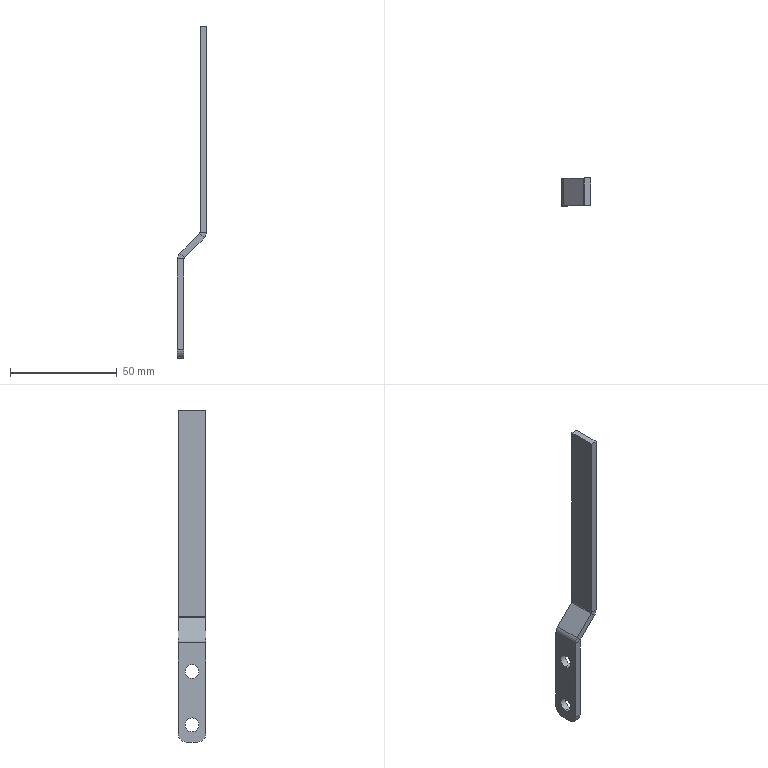Component | SolidWorks | GlassDoorAssembly-1_828LockAssembly-1_UpperPullRod-1 | 1 solid | 28 faces | box 13.61 x 13 x 155.61 mm | volume 6013 mm3 | plane 18 | cylinder 10 | commonest cylinder face diameters 6.5 x4 7.473 x2 1.473 x2 8 x2
STEP:
#1=COLOUR_RGB('',0.7922,0.8196,0.9333);
#2=FILL_AREA_STYLE_COLOUR('',#1);
#3=FILL_AREA_STYLE('',(#2));
#4=SURFACE_STYLE_FILL_AREA(#3);
#5=SURFACE_SIDE_STYLE('',(#4));
#6=SURFACE_STYLE_USAGE(.BOTH.,#5);
#7=PRESENTATION_STYLE_ASSIGNMENT((#6));
#8=CARTESIAN_POINT('',(-16.306,-19.747,-36.852));
#9=VERTEX_POINT('',#8);
#10=CARTESIAN_POINT('',(-16.306,-19.747,-36.596));
#11=VERTEX_POINT('',#10);
#12=CARTESIAN_POINT('',(-16.306,-19.747,-36.724));
#13=DIRECTION('',(1.,0.,0.));
#14=DIRECTION('',(0.,0.,1.));
#15=AXIS2_PLACEMENT_3D('',#12,#13,#14);
#16=CIRCLE('',#15,0.128);
#17=EDGE_CURVE('',#9,#11,#16,.T.);
#18=ORIENTED_EDGE('',*,*,#17,.F.);
#19=CARTESIAN_POINT('',(-16.188,-19.747,-36.852));
#20=VERTEX_POINT('',#19);
#21=CARTESIAN_POINT('',(-16.306,-19.747,-36.852));
#22=DIRECTION('',(1.,0.,0.));
#23=VECTOR('',#22,39.37);
#24=LINE('',#21,#23);
#25=EDGE_CURVE('',#9,#20,#24,.T.);
#26=ORIENTED_EDGE('',*,*,#25,.T.);
#27=CARTESIAN_POINT('',(-16.188,-19.747,-36.596));
#28=VERTEX_POINT('',#27);
#29=CARTESIAN_POINT('',(-16.188,-19.747,-36.724));
#30=DIRECTION('',(1.,0.,0.));
#31=DIRECTION('',(0.,0.,1.));
#32=AXIS2_PLACEMENT_3D('',#29,#30,#31);
#33=CIRCLE('',#32,0.128);
#34=EDGE_CURVE('',#20,#28,#33,.T.);
#35=ORIENTED_EDGE('',*,*,#34,.T.);
#36=CARTESIAN_POINT('',(-16.306,-19.747,-36.596));
#37=DIRECTION('',(1.,0.,0.));
#38=VECTOR('',#37,39.37);
#39=LINE('',#36,#38);
#40=EDGE_CURVE('',#11,#28,#39,.T.);
#41=ORIENTED_EDGE('',*,*,#40,.F.);
#42=EDGE_LOOP('',(#18,#26,#35,#41));
#43=FACE_OUTER_BOUND('',#42,.T.);
#44=CARTESIAN_POINT('',(-16.306,-19.747,-36.724));
#45=DIRECTION('',(1.,0.,0.));
#46=DIRECTION('',(0.,0.,1.));
#47=AXIS2_PLACEMENT_3D('',#44,#45,#46);
#48=CYLINDRICAL_SURFACE('',#47,0.128);
#49=ADVANCED_FACE('',(#43),#48,.F.);
#50=CARTESIAN_POINT('',(-16.306,-19.747,-37.836));
#51=VERTEX_POINT('',#50);
#52=CARTESIAN_POINT('',(-16.306,-19.747,-37.58));
#53=VERTEX_POINT('',#52);
#54=CARTESIAN_POINT('',(-16.306,-19.747,-37.708));
#55=DIRECTION('',(1.,0.,0.));
#56=DIRECTION('',(0.,0.,1.));
#57=AXIS2_PLACEMENT_3D('',#54,#55,#56);
#58=CIRCLE('',#57,0.128);
#59=EDGE_CURVE('',#51,#53,#58,.T.);
#60=ORIENTED_EDGE('',*,*,#59,.F.);
#61=CARTESIAN_POINT('',(-16.188,-19.747,-37.836));
#62=VERTEX_POINT('',#61);
#63=CARTESIAN_POINT('',(-16.306,-19.747,-37.836));
#64=DIRECTION('',(1.,0.,0.));
#65=VECTOR('',#64,39.37);
#66=LINE('',#63,#65);
#67=EDGE_CURVE('',#51,#62,#66,.T.);
#68=ORIENTED_EDGE('',*,*,#67,.T.);
#69=CARTESIAN_POINT('',(-16.188,-19.747,-37.58));
#70=VERTEX_POINT('',#69);
#71=CARTESIAN_POINT('',(-16.188,-19.747,-37.708));
#72=DIRECTION('',(1.,0.,0.));
#73=DIRECTION('',(0.,0.,1.));
#74=AXIS2_PLACEMENT_3D('',#71,#72,#73);
#75=CIRCLE('',#74,0.128);
#76=EDGE_CURVE('',#62,#70,#75,.T.);
#77=ORIENTED_EDGE('',*,*,#76,.T.);
#78=CARTESIAN_POINT('',(-16.306,-19.747,-37.58));
#79=DIRECTION('',(1.,0.,0.));
#80=VECTOR('',#79,39.37);
#81=LINE('',#78,#80);
#82=EDGE_CURVE('',#53,#70,#81,.T.);
#83=ORIENTED_EDGE('',*,*,#82,.F.);
#84=EDGE_LOOP('',(#60,#68,#77,#83));
#85=FACE_OUTER_BOUND('',#84,.T.);
#86=CARTESIAN_POINT('',(-16.306,-19.747,-37.708));
#87=DIRECTION('',(1.,0.,0.));
#88=DIRECTION('',(0.,0.,1.));
#89=AXIS2_PLACEMENT_3D('',#86,#87,#88);
#90=CYLINDRICAL_SURFACE('',#89,0.128);
#91=ADVANCED_FACE('',(#85),#90,.F.);
#92=CARTESIAN_POINT('',(-16.18,-19.491,-36.174));
#93=VERTEX_POINT('',#92);
#94=CARTESIAN_POINT('',(-16.263,-19.491,-36.09));
#95=VERTEX_POINT('',#94);
#96=CARTESIAN_POINT('',(-16.18,-19.491,-36.174));
#97=DIRECTION('',(-0.7071,-0.,0.7071));
#98=VECTOR('',#97,39.37);
#99=LINE('',#96,#98);
#100=EDGE_CURVE('',#93,#95,#99,.T.);
#101=ORIENTED_EDGE('',*,*,#100,.T.);
#102=CARTESIAN_POINT('',(-15.897,-19.491,-35.724));
#103=VERTEX_POINT('',#102);
#104=CARTESIAN_POINT('',(-15.889,-19.491,-35.716));
#105=DIRECTION('',(0.7071,0.,0.7071));
#106=VECTOR('',#105,39.37);
#107=LINE('',#104,#106);
#108=EDGE_CURVE('',#95,#103,#107,.T.);
#109=ORIENTED_EDGE('',*,*,#108,.T.);
#110=CARTESIAN_POINT('',(-15.814,-19.491,-35.808));
#111=VERTEX_POINT('',#110);
#112=CARTESIAN_POINT('',(-15.897,-19.491,-35.724));
#113=DIRECTION('',(0.7071,0.,-0.7071));
#114=VECTOR('',#113,39.37);
#115=LINE('',#112,#114);
#116=EDGE_CURVE('',#103,#111,#115,.T.);
#117=ORIENTED_EDGE('',*,*,#116,.T.);
#118=CARTESIAN_POINT('',(-15.805,-19.491,-35.799));
#119=DIRECTION('',(0.7071,0.,0.7071));
#120=VECTOR('',#119,39.37);
#121=LINE('',#118,#120);
#122=EDGE_CURVE('',#93,#111,#121,.T.);
#123=ORIENTED_EDGE('',*,*,#122,.F.);
#124=EDGE_LOOP('',(#101,#109,#117,#123));
#125=FACE_OUTER_BOUND('',#124,.T.);
#126=CARTESIAN_POINT('',(-15.805,-19.491,-35.799));
#127=DIRECTION('',(0.,-1.,-0.));
#128=DIRECTION('',(-1.,-0.,-0.));
#129=AXIS2_PLACEMENT_3D('',#126,#127,#128);
#130=PLANE('',#129);
#131=ADVANCED_FACE('',(#125),#130,.F.);
#132=CARTESIAN_POINT('',(-16.18,-20.003,-36.174));
#133=VERTEX_POINT('',#132);
#134=CARTESIAN_POINT('',(-16.263,-20.003,-36.09));
#135=VERTEX_POINT('',#134);
#136=CARTESIAN_POINT('',(-16.18,-20.003,-36.174));
#137=DIRECTION('',(-0.7071,-0.,0.7071));
#138=VECTOR('',#137,39.37);
#139=LINE('',#136,#138);
#140=EDGE_CURVE('',#133,#135,#139,.T.);
#141=ORIENTED_EDGE('',*,*,#140,.F.);
#142=CARTESIAN_POINT('',(-15.814,-20.003,-35.808));
#143=VERTEX_POINT('',#142);
#144=CARTESIAN_POINT('',(-16.188,-20.003,-36.182));
#145=DIRECTION('',(-0.7071,-0.,-0.7071));
#146=VECTOR('',#145,39.37);
#147=LINE('',#144,#146);
#148=EDGE_CURVE('',#143,#133,#147,.T.);
#149=ORIENTED_EDGE('',*,*,#148,.F.);
#150=CARTESIAN_POINT('',(-15.897,-20.003,-35.724));
#151=VERTEX_POINT('',#150);
#152=CARTESIAN_POINT('',(-15.897,-20.003,-35.724));
#153=DIRECTION('',(0.7071,0.,-0.7071));
#154=VECTOR('',#153,39.37);
#155=LINE('',#152,#154);
#156=EDGE_CURVE('',#151,#143,#155,.T.);
#157=ORIENTED_EDGE('',*,*,#156,.F.);
#158=CARTESIAN_POINT('',(-16.272,-20.003,-36.099));
#159=DIRECTION('',(-0.7071,-0.,-0.7071));
#160=VECTOR('',#159,39.37);
#161=LINE('',#158,#160);
#162=EDGE_CURVE('',#151,#135,#161,.T.);
#163=ORIENTED_EDGE('',*,*,#162,.T.);
#164=EDGE_LOOP('',(#141,#149,#157,#163));
#165=FACE_OUTER_BOUND('',#164,.T.);
#166=CARTESIAN_POINT('',(-16.188,-20.003,-36.182));
#167=DIRECTION('',(-0.,1.,0.));
#168=DIRECTION('',(1.,0.,0.));
#169=AXIS2_PLACEMENT_3D('',#166,#167,#168);
#170=PLANE('',#169);
#171=ADVANCED_FACE('',(#165),#170,.F.);
#172=CARTESIAN_POINT('',(-16.18,-19.491,-36.174));
#173=DIRECTION('',(0.,-1.,-0.));
#174=VECTOR('',#173,39.37);
#175=LINE('',#172,#174);
#176=EDGE_CURVE('',#93,#133,#175,.T.);
#177=ORIENTED_EDGE('',*,*,#176,.F.);
#178=ORIENTED_EDGE('',*,*,#122,.T.);
#179=CARTESIAN_POINT('',(-15.814,-19.491,-35.808));
#180=DIRECTION('',(-0.,1.,0.));
#181=VECTOR('',#180,39.37);
#182=LINE('',#179,#181);
#183=EDGE_CURVE('',#143,#111,#182,.T.);
#184=ORIENTED_EDGE('',*,*,#183,.F.);
#185=ORIENTED_EDGE('',*,*,#148,.T.);
#186=EDGE_LOOP('',(#177,#178,#184,#185));
#187=FACE_OUTER_BOUND('',#186,.T.);
#188=CARTESIAN_POINT('',(-16.188,-19.491,-36.182));
#189=DIRECTION('',(-0.7071,-0.,0.7071));
#190=DIRECTION('',(-0.7071,-0.,-0.7071));
#191=AXIS2_PLACEMENT_3D('',#188,#189,#190);
#192=PLANE('',#191);
#193=ADVANCED_FACE('',(#187),#192,.F.);
#194=ORIENTED_EDGE('',*,*,#108,.F.);
#195=CARTESIAN_POINT('',(-16.263,-19.491,-36.09));
#196=DIRECTION('',(0.,-1.,-0.));
#197=VECTOR('',#196,39.37);
#198=LINE('',#195,#197);
#199=EDGE_CURVE('',#95,#135,#198,.T.);
#200=ORIENTED_EDGE('',*,*,#199,.T.);
#201=ORIENTED_EDGE('',*,*,#162,.F.);
#202=CARTESIAN_POINT('',(-15.897,-19.491,-35.724));
#203=DIRECTION('',(0.,-1.,-0.));
#204=VECTOR('',#203,39.37);
#205=LINE('',#202,#204);
#206=EDGE_CURVE('',#103,#151,#205,.T.);
#207=ORIENTED_EDGE('',*,*,#206,.F.);
#208=EDGE_LOOP('',(#194,#200,#201,#207));
#209=FACE_OUTER_BOUND('',#208,.T.);
#210=CARTESIAN_POINT('',(-16.272,-19.491,-36.099));
#211=DIRECTION('',(-0.7071,-0.,0.7071));
#212=DIRECTION('',(-0.7071,-0.,-0.7071));
#213=AXIS2_PLACEMENT_3D('',#210,#211,#212);
#214=PLANE('',#213);
#215=ADVANCED_FACE('',(#209),#214,.T.);
#216=CARTESIAN_POINT('',(-15.889,-20.003,-35.704));
#217=VERTEX_POINT('',#216);
#218=CARTESIAN_POINT('',(-15.889,-20.003,-31.897));
#219=VERTEX_POINT('',#218);
#220=CARTESIAN_POINT('',(-15.889,-20.003,-31.897));
#221=DIRECTION('',(-0.,-0.,1.));
#222=VECTOR('',#221,39.37);
#223=LINE('',#220,#222);
#224=EDGE_CURVE('',#217,#219,#223,.T.);
#225=ORIENTED_EDGE('',*,*,#224,.F.);
#226=CARTESIAN_POINT('',(-15.771,-20.003,-35.704));
#227=VERTEX_POINT('',#226);
#228=CARTESIAN_POINT('',(-15.889,-20.003,-35.704));
#229=DIRECTION('',(1.,0.,0.));
#230=VECTOR('',#229,39.37);
#231=LINE('',#228,#230);
#232=EDGE_CURVE('',#217,#227,#231,.T.);
#233=ORIENTED_EDGE('',*,*,#232,.T.);
#234=CARTESIAN_POINT('',(-15.771,-20.003,-31.897));
#235=VERTEX_POINT('',#234);
#236=CARTESIAN_POINT('',(-15.771,-20.003,-31.897));
#237=DIRECTION('',(-0.,-0.,1.));
#238=VECTOR('',#237,39.37);
#239=LINE('',#236,#238);
#240=EDGE_CURVE('',#227,#235,#239,.T.);
#241=ORIENTED_EDGE('',*,*,#240,.T.);
#242=CARTESIAN_POINT('',(-15.771,-20.003,-31.897));
#243=DIRECTION('',(-1.,-0.,-0.));
#244=VECTOR('',#243,39.37);
#245=LINE('',#242,#244);
#246=EDGE_CURVE('',#235,#219,#245,.T.);
#247=ORIENTED_EDGE('',*,*,#246,.T.);
#248=EDGE_LOOP('',(#225,#233,#241,#247));
#249=FACE_OUTER_BOUND('',#248,.T.);
#250=CARTESIAN_POINT('',(-15.771,-20.003,-31.897));
#251=DIRECTION('',(0.,-1.,-0.));
#252=DIRECTION('',(-1.,-0.,-0.));
#253=AXIS2_PLACEMENT_3D('',#250,#251,#252);
#254=PLANE('',#253);
#255=ADVANCED_FACE('',(#249),#254,.T.);
#256=CARTESIAN_POINT('',(-15.771,-19.491,-35.704));
#257=VERTEX_POINT('',#256);
#258=CARTESIAN_POINT('',(-15.771,-20.003,-35.704));
#259=DIRECTION('',(-0.,1.,0.));
#260=VECTOR('',#259,39.37);
#261=LINE('',#258,#260);
#262=EDGE_CURVE('',#227,#257,#261,.T.);
#263=ORIENTED_EDGE('',*,*,#262,.T.);
#264=CARTESIAN_POINT('',(-15.771,-19.491,-31.897));
#265=VERTEX_POINT('',#264);
#266=CARTESIAN_POINT('',(-15.771,-19.491,-31.897));
#267=DIRECTION('',(0.,0.,-1.));
#268=VECTOR('',#267,39.37);
#269=LINE('',#266,#268);
#270=EDGE_CURVE('',#265,#257,#269,.T.);
#271=ORIENTED_EDGE('',*,*,#270,.F.);
#272=CARTESIAN_POINT('',(-15.771,-20.003,-31.897));
#273=DIRECTION('',(-0.,1.,0.));
#274=VECTOR('',#273,39.37);
#275=LINE('',#272,#274);
#276=EDGE_CURVE('',#235,#265,#275,.T.);
#277=ORIENTED_EDGE('',*,*,#276,.F.);
#278=ORIENTED_EDGE('',*,*,#240,.F.);
#279=EDGE_LOOP('',(#263,#271,#277,#278));
#280=FACE_OUTER_BOUND('',#279,.T.);
#281=CARTESIAN_POINT('',(-15.771,-19.491,-35.716));
#282=DIRECTION('',(-1.,-0.,-0.));
#283=DIRECTION('',(0.,0.,-1.));
#284=AXIS2_PLACEMENT_3D('',#281,#282,#283);
#285=PLANE('',#284);
#286=ADVANCED_FACE('',(#280),#285,.F.);
#287=CARTESIAN_POINT('',(-15.889,-19.491,-31.897));
#288=VERTEX_POINT('',#287);
#289=CARTESIAN_POINT('',(-15.889,-19.491,-35.704));
#290=VERTEX_POINT('',#289);
#291=CARTESIAN_POINT('',(-15.889,-19.491,-31.897));
#292=DIRECTION('',(0.,0.,-1.));
#293=VECTOR('',#292,39.37);
#294=LINE('',#291,#293);
#295=EDGE_CURVE('',#288,#290,#294,.T.);
#296=ORIENTED_EDGE('',*,*,#295,.T.);
#297=CARTESIAN_POINT('',(-15.889,-20.003,-35.704));
#298=DIRECTION('',(-0.,1.,0.));
#299=VECTOR('',#298,39.37);
#300=LINE('',#297,#299);
#301=EDGE_CURVE('',#217,#290,#300,.T.);
#302=ORIENTED_EDGE('',*,*,#301,.F.);
#303=ORIENTED_EDGE('',*,*,#224,.T.);
#304=CARTESIAN_POINT('',(-15.889,-20.003,-31.897));
#305=DIRECTION('',(-0.,1.,0.));
#306=VECTOR('',#305,39.37);
#307=LINE('',#304,#306);
#308=EDGE_CURVE('',#219,#288,#307,.T.);
#309=ORIENTED_EDGE('',*,*,#308,.T.);
#310=EDGE_LOOP('',(#296,#302,#303,#309));
#311=FACE_OUTER_BOUND('',#310,.T.);
#312=CARTESIAN_POINT('',(-15.889,-19.491,-35.716));
#313=DIRECTION('',(-1.,-0.,-0.));
#314=DIRECTION('',(0.,0.,-1.));
#315=AXIS2_PLACEMENT_3D('',#312,#313,#314);
#316=PLANE('',#315);
#317=ADVANCED_FACE('',(#311),#316,.T.);
#318=CARTESIAN_POINT('',(-15.889,-19.491,-35.704));
#319=DIRECTION('',(1.,0.,0.));
#320=VECTOR('',#319,39.37);
#321=LINE('',#318,#320);
#322=EDGE_CURVE('',#290,#257,#321,.T.);
#323=ORIENTED_EDGE('',*,*,#322,.F.);
#324=ORIENTED_EDGE('',*,*,#295,.F.);
#325=CARTESIAN_POINT('',(-15.771,-19.491,-31.897));
#326=DIRECTION('',(-1.,-0.,-0.));
#327=VECTOR('',#326,39.37);
#328=LINE('',#325,#327);
#329=EDGE_CURVE('',#265,#288,#328,.T.);
#330=ORIENTED_EDGE('',*,*,#329,.F.);
#331=ORIENTED_EDGE('',*,*,#270,.T.);
#332=EDGE_LOOP('',(#323,#324,#330,#331));
#333=FACE_OUTER_BOUND('',#332,.T.);
#334=CARTESIAN_POINT('',(-15.771,-19.491,-31.897));
#335=DIRECTION('',(-0.,1.,0.));
#336=DIRECTION('',(1.,0.,0.));
#337=AXIS2_PLACEMENT_3D('',#334,#335,#336);
#338=PLANE('',#337);
#339=ADVANCED_FACE('',(#333),#338,.T.);
#340=ORIENTED_EDGE('',*,*,#308,.F.);
#341=ORIENTED_EDGE('',*,*,#246,.F.);
#342=ORIENTED_EDGE('',*,*,#276,.T.);
#343=ORIENTED_EDGE('',*,*,#329,.T.);
#344=EDGE_LOOP('',(#340,#341,#342,#343));
#345=FACE_OUTER_BOUND('',#344,.T.);
#346=CARTESIAN_POINT('',(-15.771,-20.003,-31.897));
#347=DIRECTION('',(-0.,-0.,1.));
#348=DIRECTION('',(-1.,-0.,-0.));
#349=AXIS2_PLACEMENT_3D('',#346,#347,#348);
#350=PLANE('',#349);
#351=ADVANCED_FACE('',(#345),#350,.T.);
#352=ORIENTED_EDGE('',*,*,#116,.F.);
#353=CARTESIAN_POINT('',(-15.918,-19.491,-35.704));
#354=DIRECTION('',(-0.,1.,0.));
#355=DIRECTION('',(-1.,0.,0.));
#356=AXIS2_PLACEMENT_3D('',#353,#354,#355);
#357=CIRCLE('',#356,0.029);
#358=EDGE_CURVE('',#290,#103,#357,.T.);
#359=ORIENTED_EDGE('',*,*,#358,.F.);
#360=ORIENTED_EDGE('',*,*,#322,.T.);
#361=CARTESIAN_POINT('',(-15.918,-19.491,-35.704));
#362=DIRECTION('',(-0.,1.,0.));
#363=DIRECTION('',(-1.,0.,-0.));
#364=AXIS2_PLACEMENT_3D('',#361,#362,#363);
#365=CIRCLE('',#364,0.1471);
#366=EDGE_CURVE('',#257,#111,#365,.T.);
#367=ORIENTED_EDGE('',*,*,#366,.T.);
#368=EDGE_LOOP('',(#352,#359,#360,#367));
#369=FACE_OUTER_BOUND('',#368,.T.);
#370=CARTESIAN_POINT('',(-15.918,-19.491,-35.704));
#371=DIRECTION('',(-0.,1.,0.));
#372=DIRECTION('',(1.,0.,0.));
#373=AXIS2_PLACEMENT_3D('',#370,#371,#372);
#374=PLANE('',#373);
#375=ADVANCED_FACE('',(#369),#374,.T.);
#376=CARTESIAN_POINT('',(-15.918,-20.003,-35.704));
#377=DIRECTION('',(0.,-1.,-0.));
#378=DIRECTION('',(-1.,0.,0.));
#379=AXIS2_PLACEMENT_3D('',#376,#377,#378);
#380=CIRCLE('',#379,0.029);
#381=EDGE_CURVE('',#151,#217,#380,.T.);
#382=ORIENTED_EDGE('',*,*,#381,.F.);
#383=ORIENTED_EDGE('',*,*,#156,.T.);
#384=CARTESIAN_POINT('',(-15.918,-20.003,-35.704));
#385=DIRECTION('',(0.,-1.,-0.));
#386=DIRECTION('',(-1.,0.,0.));
#387=AXIS2_PLACEMENT_3D('',#384,#385,#386);
#388=CIRCLE('',#387,0.1471);
#389=EDGE_CURVE('',#143,#227,#388,.T.);
#390=ORIENTED_EDGE('',*,*,#389,.T.);
#391=ORIENTED_EDGE('',*,*,#232,.F.);
#392=EDGE_LOOP('',(#382,#383,#390,#391));
#393=FACE_OUTER_BOUND('',#392,.T.);
#394=CARTESIAN_POINT('',(-15.918,-20.003,-35.704));
#395=DIRECTION('',(-0.,1.,0.));
#396=DIRECTION('',(1.,0.,0.));
#397=AXIS2_PLACEMENT_3D('',#394,#395,#396);
#398=PLANE('',#397);
#399=ADVANCED_FACE('',(#393),#398,.F.);
#400=ORIENTED_EDGE('',*,*,#262,.F.);
#401=ORIENTED_EDGE('',*,*,#389,.F.);
#402=ORIENTED_EDGE('',*,*,#183,.T.);
#403=ORIENTED_EDGE('',*,*,#366,.F.);
#404=EDGE_LOOP('',(#400,#401,#402,#403));
#405=FACE_OUTER_BOUND('',#404,.T.);
#406=CARTESIAN_POINT('',(-15.918,-20.003,-35.704));
#407=DIRECTION('',(0.,-1.,-0.));
#408=DIRECTION('',(0.7071,0.,-0.7071));
#409=AXIS2_PLACEMENT_3D('',#406,#407,#408);
#410=CYLINDRICAL_SURFACE('',#409,0.1471);
#411=ADVANCED_FACE('',(#405),#410,.T.);
#412=ORIENTED_EDGE('',*,*,#301,.T.);
#413=ORIENTED_EDGE('',*,*,#358,.T.);
#414=ORIENTED_EDGE('',*,*,#206,.T.);
#415=ORIENTED_EDGE('',*,*,#381,.T.);
#416=EDGE_LOOP('',(#412,#413,#414,#415));
#417=FACE_OUTER_BOUND('',#416,.T.);
#418=CARTESIAN_POINT('',(-15.918,-20.003,-35.704));
#419=DIRECTION('',(0.,-1.,-0.));
#420=DIRECTION('',(0.7071,0.,-0.7071));
#421=AXIS2_PLACEMENT_3D('',#418,#419,#420);
#422=CYLINDRICAL_SURFACE('',#421,0.029);
#423=ADVANCED_FACE('',(#417),#422,.F.);
#424=CARTESIAN_POINT('',(-16.188,-20.003,-36.194));
#425=VERTEX_POINT('',#424);
#426=CARTESIAN_POINT('',(-16.306,-20.003,-36.194));
#427=VERTEX_POINT('',#426);
#428=CARTESIAN_POINT('',(-16.188,-20.003,-36.194));
#429=DIRECTION('',(-1.,-0.,-0.));
#430=VECTOR('',#429,39.37);
#431=LINE('',#428,#430);
#432=EDGE_CURVE('',#425,#427,#431,.T.);
#433=ORIENTED_EDGE('',*,*,#432,.F.);
#434=CARTESIAN_POINT('',(-16.159,-20.003,-36.194));
#435=DIRECTION('',(0.,-1.,-0.));
#436=DIRECTION('',(1.,0.,0.));
#437=AXIS2_PLACEMENT_3D('',#434,#435,#436);
#438=CIRCLE('',#437,0.029);
#439=EDGE_CURVE('',#133,#425,#438,.T.);
#440=ORIENTED_EDGE('',*,*,#439,.F.);
#441=ORIENTED_EDGE('',*,*,#140,.T.);
#442=CARTESIAN_POINT('',(-16.159,-20.003,-36.194));
#443=DIRECTION('',(0.,-1.,-0.));
#444=DIRECTION('',(1.,0.,0.));
#445=AXIS2_PLACEMENT_3D('',#442,#443,#444);
#446=CIRCLE('',#445,0.1471);
#447=EDGE_CURVE('',#135,#427,#446,.T.);
#448=ORIENTED_EDGE('',*,*,#447,.T.);
#449=EDGE_LOOP('',(#433,#440,#441,#448));
#450=FACE_OUTER_BOUND('',#449,.T.);
#451=CARTESIAN_POINT('',(-16.159,-20.003,-36.194));
#452=DIRECTION('',(0.,-1.,-0.));
#453=DIRECTION('',(-1.,-0.,-0.));
#454=AXIS2_PLACEMENT_3D('',#451,#452,#453);
#455=PLANE('',#454);
#456=ADVANCED_FACE('',(#450),#455,.T.);
#457=CARTESIAN_POINT('',(-16.188,-19.491,-36.194));
#458=VERTEX_POINT('',#457);
#459=CARTESIAN_POINT('',(-16.159,-19.491,-36.194));
#460=DIRECTION('',(-0.,1.,0.));
#461=DIRECTION('',(1.,0.,0.));
#462=AXIS2_PLACEMENT_3D('',#459,#460,#461);
#463=CIRCLE('',#462,0.029);
#464=EDGE_CURVE('',#458,#93,#463,.T.);
#465=ORIENTED_EDGE('',*,*,#464,.F.);
#466=CARTESIAN_POINT('',(-16.306,-19.491,-36.194));
#467=VERTEX_POINT('',#466);
#468=CARTESIAN_POINT('',(-16.188,-19.491,-36.194));
#469=DIRECTION('',(-1.,-0.,-0.));
#470=VECTOR('',#469,39.37);
#471=LINE('',#468,#470);
#472=EDGE_CURVE('',#458,#467,#471,.T.);
#473=ORIENTED_EDGE('',*,*,#472,.T.);
#474=CARTESIAN_POINT('',(-16.159,-19.491,-36.194));
#475=DIRECTION('',(-0.,1.,0.));
#476=DIRECTION('',(1.,0.,0.));
#477=AXIS2_PLACEMENT_3D('',#474,#475,#476);
#478=CIRCLE('',#477,0.1471);
#479=EDGE_CURVE('',#467,#95,#478,.T.);
#480=ORIENTED_EDGE('',*,*,#479,.T.);
#481=ORIENTED_EDGE('',*,*,#100,.F.);
#482=EDGE_LOOP('',(#465,#473,#480,#481));
#483=FACE_OUTER_BOUND('',#482,.T.);
#484=CARTESIAN_POINT('',(-16.159,-19.491,-36.194));
#485=DIRECTION('',(0.,-1.,-0.));
#486=DIRECTION('',(-1.,-0.,-0.));
#487=AXIS2_PLACEMENT_3D('',#484,#485,#486);
#488=PLANE('',#487);
#489=ADVANCED_FACE('',(#483),#488,.F.);
#490=ORIENTED_EDGE('',*,*,#199,.F.);
#491=ORIENTED_EDGE('',*,*,#479,.F.);
#492=CARTESIAN_POINT('',(-16.306,-19.491,-36.194));
#493=DIRECTION('',(-0.,1.,0.));
#494=VECTOR('',#493,39.37);
#495=LINE('',#492,#494);
#496=EDGE_CURVE('',#427,#467,#495,.T.);
#497=ORIENTED_EDGE('',*,*,#496,.F.);
#498=ORIENTED_EDGE('',*,*,#447,.F.);
#499=EDGE_LOOP('',(#490,#491,#497,#498));
#500=FACE_OUTER_BOUND('',#499,.T.);
#501=CARTESIAN_POINT('',(-16.159,-19.491,-36.194));
#502=DIRECTION('',(-0.,1.,0.));
#503=DIRECTION('',(-1.,0.,0.));
#504=AXIS2_PLACEMENT_3D('',#501,#502,#503);
#505=CYLINDRICAL_SURFACE('',#504,0.1471);
#506=ADVANCED_FACE('',(#500),#505,.T.);
#507=ORIENTED_EDGE('',*,*,#176,.T.);
#508=ORIENTED_EDGE('',*,*,#439,.T.);
#509=CARTESIAN_POINT('',(-16.188,-20.003,-36.194));
#510=DIRECTION('',(-0.,1.,0.));
#511=VECTOR('',#510,39.37);
#512=LINE('',#509,#511);
#513=EDGE_CURVE('',#425,#458,#512,.T.);
#514=ORIENTED_EDGE('',*,*,#513,.T.);
#515=ORIENTED_EDGE('',*,*,#464,.T.);
#516=EDGE_LOOP('',(#507,#508,#514,#515));
#517=FACE_OUTER_BOUND('',#516,.T.);
#518=CARTESIAN_POINT('',(-16.159,-19.491,-36.194));
#519=DIRECTION('',(-0.,1.,0.));
#520=DIRECTION('',(-1.,0.,0.));
#521=AXIS2_PLACEMENT_3D('',#518,#519,#520);
#522=CYLINDRICAL_SURFACE('',#521,0.029);
#523=ADVANCED_FACE('',(#517),#522,.F.);
#524=CARTESIAN_POINT('',(-16.188,-19.491,-37.865));
#525=VERTEX_POINT('',#524);
#526=CARTESIAN_POINT('',(-16.188,-19.491,-36.182));
#527=DIRECTION('',(-0.,-0.,1.));
#528=VECTOR('',#527,39.37);
#529=LINE('',#526,#528);
#530=EDGE_CURVE('',#525,#458,#529,.T.);
#531=ORIENTED_EDGE('',*,*,#530,.F.);
#532=CARTESIAN_POINT('',(-16.306,-19.491,-37.865));
#533=VERTEX_POINT('',#532);
#534=CARTESIAN_POINT('',(-16.306,-19.491,-37.865));
#535=DIRECTION('',(-1.,-0.,-0.));
#536=VECTOR('',#535,39.37);
#537=LINE('',#534,#536);
#538=EDGE_CURVE('',#525,#533,#537,.T.);
#539=ORIENTED_EDGE('',*,*,#538,.T.);
#540=CARTESIAN_POINT('',(-16.306,-19.491,-36.182));
#541=DIRECTION('',(-0.,-0.,1.));
#542=VECTOR('',#541,39.37);
#543=LINE('',#540,#542);
#544=EDGE_CURVE('',#533,#467,#543,.T.);
#545=ORIENTED_EDGE('',*,*,#544,.T.);
#546=ORIENTED_EDGE('',*,*,#472,.F.);
#547=EDGE_LOOP('',(#531,#539,#545,#546));
#548=FACE_OUTER_BOUND('',#547,.T.);
#549=CARTESIAN_POINT('',(-16.306,-19.491,-36.182));
#550=DIRECTION('',(-0.,1.,0.));
#551=DIRECTION('',(1.,0.,0.));
#552=AXIS2_PLACEMENT_3D('',#549,#550,#551);
#553=PLANE('',#552);
#554=ADVANCED_FACE('',(#548),#553,.T.);
#555=CARTESIAN_POINT('',(-16.306,-20.003,-37.865));
#556=VERTEX_POINT('',#555);
#557=CARTESIAN_POINT('',(-16.306,-20.003,-38.023));
#558=DIRECTION('',(0.,0.,-1.));
#559=VECTOR('',#558,39.37);
#560=LINE('',#557,#559);
#561=EDGE_CURVE('',#427,#556,#560,.T.);
#562=ORIENTED_EDGE('',*,*,#561,.T.);
#563=CARTESIAN_POINT('',(-16.188,-20.003,-37.865));
#564=VERTEX_POINT('',#563);
#565=CARTESIAN_POINT('',(-16.306,-20.003,-37.865));
#566=DIRECTION('',(1.,0.,0.));
#567=VECTOR('',#566,39.37);
#568=LINE('',#565,#567);
#569=EDGE_CURVE('',#556,#564,#568,.T.);
#570=ORIENTED_EDGE('',*,*,#569,.T.);
#571=CARTESIAN_POINT('',(-16.188,-20.003,-38.023));
#572=DIRECTION('',(0.,0.,-1.));
#573=VECTOR('',#572,39.37);
#574=LINE('',#571,#573);
#575=EDGE_CURVE('',#425,#564,#574,.T.);
#576=ORIENTED_EDGE('',*,*,#575,.F.);
#577=ORIENTED_EDGE('',*,*,#432,.T.);
#578=EDGE_LOOP('',(#562,#570,#576,#577));
#579=FACE_OUTER_BOUND('',#578,.T.);
#580=CARTESIAN_POINT('',(-16.306,-20.003,-38.023));
#581=DIRECTION('',(0.,-1.,-0.));
#582=DIRECTION('',(-1.,-0.,-0.));
#583=AXIS2_PLACEMENT_3D('',#580,#581,#582);
#584=PLANE('',#583);
#585=ADVANCED_FACE('',(#579),#584,.T.);
#586=CARTESIAN_POINT('',(-16.306,-19.747,-36.724));
#587=DIRECTION('',(1.,0.,0.));
#588=DIRECTION('',(0.,0.,1.));
#589=AXIS2_PLACEMENT_3D('',#586,#587,#588);
#590=CIRCLE('',#589,0.128);
#591=EDGE_CURVE('',#11,#9,#590,.T.);
#592=ORIENTED_EDGE('',*,*,#591,.T.);
#593=ORIENTED_EDGE('',*,*,#17,.T.);
#594=EDGE_LOOP('',(#592,#593));
#595=FACE_BOUND('',#594,.T.);
#596=CARTESIAN_POINT('',(-16.306,-19.747,-37.708));
#597=DIRECTION('',(1.,0.,0.));
#598=DIRECTION('',(0.,0.,1.));
#599=AXIS2_PLACEMENT_3D('',#596,#597,#598);
#600=CIRCLE('',#599,0.128);
#601=EDGE_CURVE('',#53,#51,#600,.T.);
#602=ORIENTED_EDGE('',*,*,#601,.T.);
#603=ORIENTED_EDGE('',*,*,#59,.T.);
#604=EDGE_LOOP('',(#602,#603));
#605=FACE_BOUND('',#604,.T.);
#606=ORIENTED_EDGE('',*,*,#544,.F.);
#607=CARTESIAN_POINT('',(-16.306,-19.649,-38.023));
#608=VERTEX_POINT('',#607);
#609=CARTESIAN_POINT('',(-16.306,-19.649,-37.865));
#610=DIRECTION('',(-1.,-0.,-0.));
#611=DIRECTION('',(0.,0.,-1.));
#612=AXIS2_PLACEMENT_3D('',#609,#610,#611);
#613=CIRCLE('',#612,0.1575);
#614=EDGE_CURVE('',#533,#608,#613,.T.);
#615=ORIENTED_EDGE('',*,*,#614,.T.);
#616=CARTESIAN_POINT('',(-16.306,-19.846,-38.023));
#617=VERTEX_POINT('',#616);
#618=CARTESIAN_POINT('',(-16.306,-19.491,-38.023));
#619=DIRECTION('',(-0.,1.,0.));
#620=VECTOR('',#619,39.37);
#621=LINE('',#618,#620);
#622=EDGE_CURVE('',#617,#608,#621,.T.);
#623=ORIENTED_EDGE('',*,*,#622,.F.);
#624=CARTESIAN_POINT('',(-16.306,-19.846,-37.865));
#625=DIRECTION('',(-1.,-0.,-0.));
#626=DIRECTION('',(0.,0.,-1.));
#627=AXIS2_PLACEMENT_3D('',#624,#625,#626);
#628=CIRCLE('',#627,0.1575);
#629=EDGE_CURVE('',#617,#556,#628,.T.);
#630=ORIENTED_EDGE('',*,*,#629,.T.);
#631=ORIENTED_EDGE('',*,*,#561,.F.);
#632=ORIENTED_EDGE('',*,*,#496,.T.);
#633=EDGE_LOOP('',(#606,#615,#623,#630,#631,#632));
#634=FACE_OUTER_BOUND('',#633,.T.);
#635=CARTESIAN_POINT('',(-16.306,-19.491,-36.182));
#636=DIRECTION('',(-1.,-0.,-0.));
#637=DIRECTION('',(0.,0.,-1.));
#638=AXIS2_PLACEMENT_3D('',#635,#636,#637);
#639=PLANE('',#638);
#640=ADVANCED_FACE('',(#595,#605,#634),#639,.T.);
#641=CARTESIAN_POINT('',(-16.188,-19.747,-36.724));
#642=DIRECTION('',(1.,0.,0.));
#643=DIRECTION('',(0.,0.,1.));
#644=AXIS2_PLACEMENT_3D('',#641,#642,#643);
#645=CIRCLE('',#644,0.128);
#646=EDGE_CURVE('',#28,#20,#645,.T.);
#647=ORIENTED_EDGE('',*,*,#646,.F.);
#648=ORIENTED_EDGE('',*,*,#34,.F.);
#649=EDGE_LOOP('',(#647,#648));
#650=FACE_BOUND('',#649,.T.);
#651=CARTESIAN_POINT('',(-16.188,-19.747,-37.708));
#652=DIRECTION('',(1.,0.,0.));
#653=DIRECTION('',(0.,0.,1.));
#654=AXIS2_PLACEMENT_3D('',#651,#652,#653);
#655=CIRCLE('',#654,0.128);
#656=EDGE_CURVE('',#70,#62,#655,.T.);
#657=ORIENTED_EDGE('',*,*,#656,.F.);
#658=ORIENTED_EDGE('',*,*,#76,.F.);
#659=EDGE_LOOP('',(#657,#658));
#660=FACE_BOUND('',#659,.T.);
#661=CARTESIAN_POINT('',(-16.188,-19.846,-38.023));
#662=VERTEX_POINT('',#661);
#663=CARTESIAN_POINT('',(-16.188,-19.649,-38.023));
#664=VERTEX_POINT('',#663);
#665=CARTESIAN_POINT('',(-16.188,-19.491,-38.023));
#666=DIRECTION('',(-0.,1.,0.));
#667=VECTOR('',#666,39.37);
#668=LINE('',#665,#667);
#669=EDGE_CURVE('',#662,#664,#668,.T.);
#670=ORIENTED_EDGE('',*,*,#669,.T.);
#671=CARTESIAN_POINT('',(-16.188,-19.649,-37.865));
#672=DIRECTION('',(1.,0.,0.));
#673=DIRECTION('',(0.,0.,-1.));
#674=AXIS2_PLACEMENT_3D('',#671,#672,#673);
#675=CIRCLE('',#674,0.1575);
#676=EDGE_CURVE('',#664,#525,#675,.T.);
#677=ORIENTED_EDGE('',*,*,#676,.T.);
#678=ORIENTED_EDGE('',*,*,#530,.T.);
#679=ORIENTED_EDGE('',*,*,#513,.F.);
#680=ORIENTED_EDGE('',*,*,#575,.T.);
#681=CARTESIAN_POINT('',(-16.188,-19.846,-37.865));
#682=DIRECTION('',(1.,0.,0.));
#683=DIRECTION('',(0.,0.,-1.));
#684=AXIS2_PLACEMENT_3D('',#681,#682,#683);
#685=CIRCLE('',#684,0.1575);
#686=EDGE_CURVE('',#564,#662,#685,.T.);
#687=ORIENTED_EDGE('',*,*,#686,.T.);
#688=EDGE_LOOP('',(#670,#677,#678,#679,#680,#687));
#689=FACE_OUTER_BOUND('',#688,.T.);
#690=CARTESIAN_POINT('',(-16.188,-19.491,-36.182));
#691=DIRECTION('',(-1.,-0.,-0.));
#692=DIRECTION('',(0.,0.,-1.));
#693=AXIS2_PLACEMENT_3D('',#690,#691,#692);
#694=PLANE('',#693);
#695=ADVANCED_FACE('',(#650,#660,#689),#694,.F.);
#696=ORIENTED_EDGE('',*,*,#622,.T.);
#697=CARTESIAN_POINT('',(-16.306,-19.649,-38.023));
#698=DIRECTION('',(1.,0.,0.));
#699=VECTOR('',#698,39.37);
#700=LINE('',#697,#699);
#701=EDGE_CURVE('',#608,#664,#700,.T.);
#702=ORIENTED_EDGE('',*,*,#701,.T.);
#703=ORIENTED_EDGE('',*,*,#669,.F.);
#704=CARTESIAN_POINT('',(-16.306,-19.846,-38.023));
#705=DIRECTION('',(-1.,-0.,-0.));
#706=VECTOR('',#705,39.37);
#707=LINE('',#704,#706);
#708=EDGE_CURVE('',#662,#617,#707,.T.);
#709=ORIENTED_EDGE('',*,*,#708,.T.);
#710=EDGE_LOOP('',(#696,#702,#703,#709));
#711=FACE_OUTER_BOUND('',#710,.T.);
#712=CARTESIAN_POINT('',(-16.306,-19.491,-38.023));
#713=DIRECTION('',(0.,0.,-1.));
#714=DIRECTION('',(1.,0.,0.));
#715=AXIS2_PLACEMENT_3D('',#712,#713,#714);
#716=PLANE('',#715);
#717=ADVANCED_FACE('',(#711),#716,.T.);
#718=ORIENTED_EDGE('',*,*,#67,.F.);
#719=ORIENTED_EDGE('',*,*,#601,.F.);
#720=ORIENTED_EDGE('',*,*,#82,.T.);
#721=ORIENTED_EDGE('',*,*,#656,.T.);
#722=EDGE_LOOP('',(#718,#719,#720,#721));
#723=FACE_OUTER_BOUND('',#722,.T.);
#724=CARTESIAN_POINT('',(-16.306,-19.747,-37.708));
#725=DIRECTION('',(1.,0.,0.));
#726=DIRECTION('',(0.,0.,1.));
#727=AXIS2_PLACEMENT_3D('',#724,#725,#726);
#728=CYLINDRICAL_SURFACE('',#727,0.128);
#729=ADVANCED_FACE('',(#723),#728,.F.);
#730=ORIENTED_EDGE('',*,*,#25,.F.);
#731=ORIENTED_EDGE('',*,*,#591,.F.);
#732=ORIENTED_EDGE('',*,*,#40,.T.);
#733=ORIENTED_EDGE('',*,*,#646,.T.);
#734=EDGE_LOOP('',(#730,#731,#732,#733));
#735=FACE_OUTER_BOUND('',#734,.T.);
#736=CARTESIAN_POINT('',(-16.306,-19.747,-36.724));
#737=DIRECTION('',(1.,0.,0.));
#738=DIRECTION('',(0.,0.,1.));
#739=AXIS2_PLACEMENT_3D('',#736,#737,#738);
#740=CYLINDRICAL_SURFACE('',#739,0.128);
#741=ADVANCED_FACE('',(#735),#740,.F.);
#742=ORIENTED_EDGE('',*,*,#614,.F.);
#743=ORIENTED_EDGE('',*,*,#538,.F.);
#744=ORIENTED_EDGE('',*,*,#676,.F.);
#745=ORIENTED_EDGE('',*,*,#701,.F.);
#746=EDGE_LOOP('',(#742,#743,#744,#745));
#747=FACE_OUTER_BOUND('',#746,.T.);
#748=CARTESIAN_POINT('',(-16.306,-19.649,-37.865));
#749=DIRECTION('',(1.,0.,0.));
#750=DIRECTION('',(0.,0.,1.));
#751=AXIS2_PLACEMENT_3D('',#748,#749,#750);
#752=CYLINDRICAL_SURFACE('',#751,0.1575);
#753=ADVANCED_FACE('',(#747),#752,.T.);
#754=ORIENTED_EDGE('',*,*,#629,.F.);
#755=ORIENTED_EDGE('',*,*,#708,.F.);
#756=ORIENTED_EDGE('',*,*,#686,.F.);
#757=ORIENTED_EDGE('',*,*,#569,.F.);
#758=EDGE_LOOP('',(#754,#755,#756,#757));
#759=FACE_OUTER_BOUND('',#758,.T.);
#760=CARTESIAN_POINT('',(-16.306,-19.846,-37.865));
#761=DIRECTION('',(1.,0.,0.));
#762=DIRECTION('',(0.,0.,1.));
#763=AXIS2_PLACEMENT_3D('',#760,#761,#762);
#764=CYLINDRICAL_SURFACE('',#763,0.1575);
#765=ADVANCED_FACE('',(#759),#764,.T.);
#766=CLOSED_SHELL('',(#49,#91,#131,#171,#193,#215,#255,#286,#317,#339,#351,#375,#399,#411,#423,#456,#489,#506,#523,#554,#585,#640,#695,#717,#729,#741,#753,#765));
#767=MANIFOLD_SOLID_BREP('',#766);
#768=STYLED_ITEM('',(#7),#767);
#769=PRESENTATION_LAYER_ASSIGNMENT('','',(#768));
#770=(LENGTH_UNIT()NAMED_UNIT(*)SI_UNIT($,.METRE.));
#771=LENGTH_MEASURE_WITH_UNIT(LENGTH_MEASURE(0.0254),#770);
#772=DIMENSIONAL_EXPONENTS(1.,0.,0.,0.,0.,0.,0.);
#773=(CONVERSION_BASED_UNIT('',#771)LENGTH_UNIT()NAMED_UNIT(#772));
#774=UNCERTAINTY_MEASURE_WITH_UNIT(LENGTH_MEASURE(0.00001),#773,'','');
#775=(NAMED_UNIT(*)PLANE_ANGLE_UNIT()SI_UNIT($,.RADIAN.));
#776=(NAMED_UNIT(*)SI_UNIT($,.STERADIAN.)SOLID_ANGLE_UNIT());
#777=(GEOMETRIC_REPRESENTATION_CONTEXT(3)GLOBAL_UNCERTAINTY_ASSIGNED_CONTEXT((#774))GLOBAL_UNIT_ASSIGNED_CONTEXT((#773,#775,#776))REPRESENTATION_CONTEXT('',''));
#778=MECHANICAL_DESIGN_GEOMETRIC_PRESENTATION_REPRESENTATION('',(#768),#777);
#779=CARTESIAN_POINT('',(0.,0.,0.));
#780=DIRECTION('',(0.,0.,1.));
#781=DIRECTION('',(1.,0.,0.));
#782=AXIS2_PLACEMENT_3D('',#779,#780,#781);
#783=(LENGTH_UNIT()NAMED_UNIT(*)SI_UNIT($,.METRE.));
#784=LENGTH_MEASURE_WITH_UNIT(LENGTH_MEASURE(0.0254),#783);
#785=DIMENSIONAL_EXPONENTS(1.,0.,0.,0.,0.,0.,0.);
#786=(CONVERSION_BASED_UNIT('',#784)LENGTH_UNIT()NAMED_UNIT(#785));
#787=UNCERTAINTY_MEASURE_WITH_UNIT(LENGTH_MEASURE(0.00001),#786,'','');
#788=(NAMED_UNIT(*)PLANE_ANGLE_UNIT()SI_UNIT($,.RADIAN.));
#789=(NAMED_UNIT(*)SI_UNIT($,.STERADIAN.)SOLID_ANGLE_UNIT());
#790=(GEOMETRIC_REPRESENTATION_CONTEXT(3)GLOBAL_UNCERTAINTY_ASSIGNED_CONTEXT((#787))GLOBAL_UNIT_ASSIGNED_CONTEXT((#786,#788,#789))REPRESENTATION_CONTEXT('',''));
#791=ADVANCED_BREP_SHAPE_REPRESENTATION('',(#767,#782),#790);